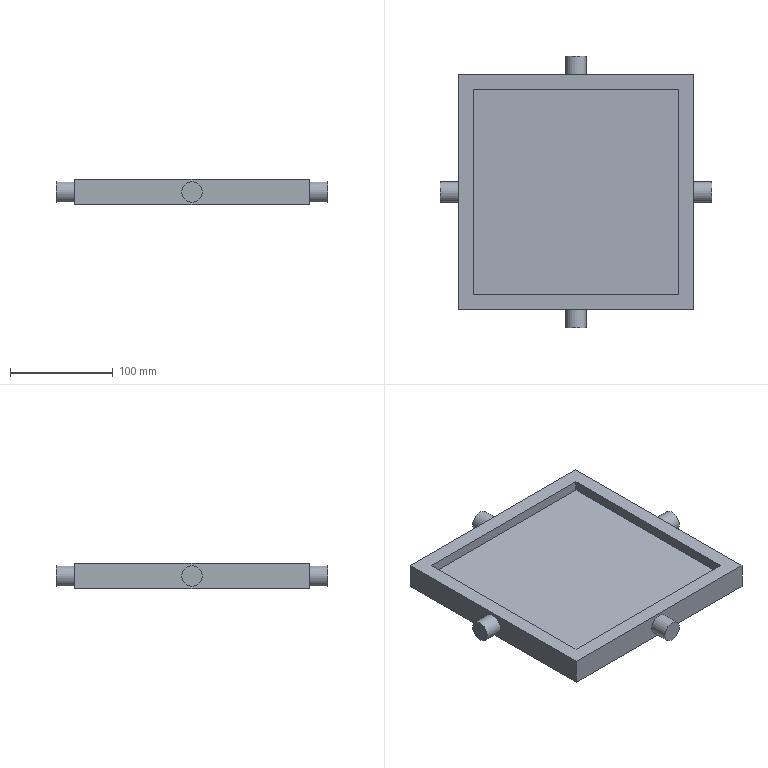Component | NX | MODEL4 | 5 solids | 23 faces | volume 933644 mm3 | plane 19 | cylinder 4 | commonest cylinder face diameters 20 x4